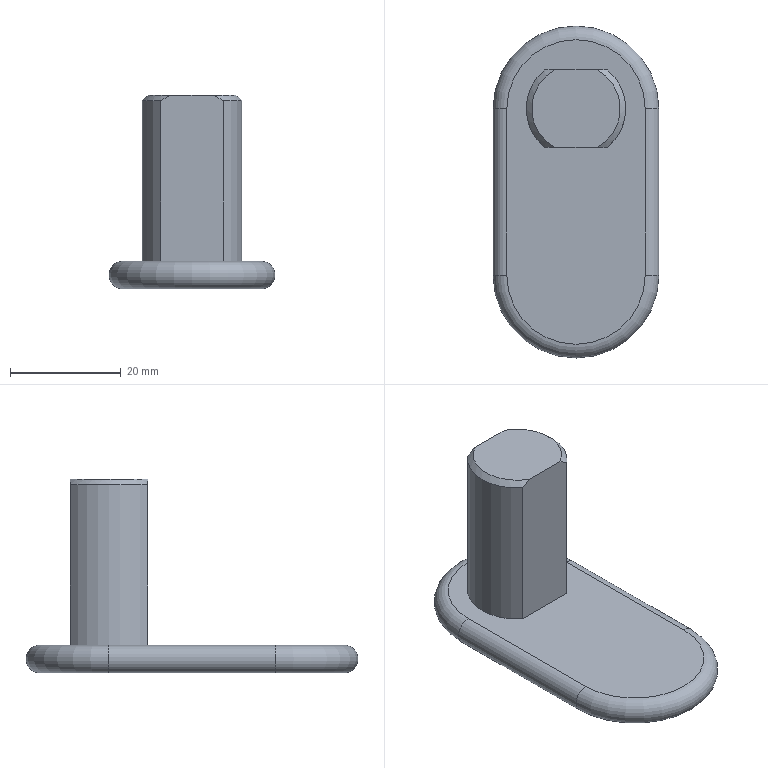Component | NX | LOWER_MOUNT | 1 solid | 13 faces | box 30 x 60 x 35 mm | volume 14320 mm3 | plane 5 | cylinder 4 | cone 2 | torus 2 | commonest cylinder face diameters 18 x2 5 x2
STEP:
#1=CARTESIAN_POINT('',(0.,0.,0.));
#2=DIRECTION('',(0.,0.,1.));
#3=DIRECTION('',(1.,0.,0.));
#4=AXIS2_PLACEMENT_3D('',#1,#2,#3);
#5=CARTESIAN_POINT('',(-12.5,94.875,-210.));
#6=VERTEX_POINT('',#5);
#7=CARTESIAN_POINT('',(12.5,94.875,-210.));
#8=VERTEX_POINT('',#7);
#9=CARTESIAN_POINT('',(0.,94.875,-210.));
#10=DIRECTION('',(0.,0.,1.));
#11=DIRECTION('',(0.,1.,0.));
#12=AXIS2_PLACEMENT_3D('',#9,#10,#11);
#13=CIRCLE('',#12,12.5);
#14=CARTESIAN_POINT('',(0.,94.875,-210.));
#15=DIRECTION('',(0.,0.,1.));
#16=DIRECTION('',(0.,1.,0.));
#17=AXIS2_PLACEMENT_3D('',#14,#15,#16);
#18=PLANE('',#17);
#19=CARTESIAN_POINT('',(0.,0.));
#20=DIRECTION('',(1.,0.));
#21=AXIS2_PLACEMENT_2D('',#19,#20);
#22=CIRCLE('',#21,12.5);
#23=(GEOMETRIC_REPRESENTATION_CONTEXT(2)PARAMETRIC_REPRESENTATION_CONTEXT()REPRESENTATION_CONTEXT('',''));
#24=DEFINITIONAL_REPRESENTATION('',(#22),#23);
#25=PCURVE('',#18,#24);
#26=CARTESIAN_POINT('',(0.,94.875,-212.5));
#27=DIRECTION('',(0.,0.,1.));
#28=DIRECTION('',(0.,1.,0.));
#29=AXIS2_PLACEMENT_3D('',#26,#27,#28);
#30=TOROIDAL_SURFACE('',#29,12.5,2.5);
#31=CARTESIAN_POINT('',(0.,7.854));
#32=DIRECTION('',(1.,0.));
#33=VECTOR('',#32,1.);
#34=LINE('',#31,#33);
#35=(GEOMETRIC_REPRESENTATION_CONTEXT(2)PARAMETRIC_REPRESENTATION_CONTEXT()REPRESENTATION_CONTEXT('',''));
#36=DEFINITIONAL_REPRESENTATION('',(#34),#35);
#37=PCURVE('',#30,#36);
#38=SURFACE_CURVE('',#13,(#25,#37),.PCURVE_S1.);
#39=EDGE_CURVE('',#6,#8,#38,.T.);
#40=ORIENTED_EDGE('',*,*,#39,.T.);
#41=CARTESIAN_POINT('',(12.5,124.875,-210.));
#42=VERTEX_POINT('',#41);
#43=CARTESIAN_POINT('',(12.5,94.875,-210.));
#44=DIRECTION('',(0.,1.,0.));
#45=VECTOR('',#44,1.);
#46=LINE('',#43,#45);
#47=CARTESIAN_POINT('',(0.,-12.5));
#48=DIRECTION('',(1.,0.));
#49=VECTOR('',#48,1.);
#50=LINE('',#47,#49);
#51=(GEOMETRIC_REPRESENTATION_CONTEXT(2)PARAMETRIC_REPRESENTATION_CONTEXT()REPRESENTATION_CONTEXT('',''));
#52=DEFINITIONAL_REPRESENTATION('',(#50),#51);
#53=PCURVE('',#18,#52);
#54=CARTESIAN_POINT('',(12.5,94.875,-212.5));
#55=DIRECTION('',(0.,-1.,0.));
#56=DIRECTION('',(0.,0.,1.));
#57=AXIS2_PLACEMENT_3D('',#54,#55,#56);
#58=CYLINDRICAL_SURFACE('',#57,2.5);
#59=CARTESIAN_POINT('',(6.283,0.));
#60=DIRECTION('',(0.,-1.));
#61=VECTOR('',#60,1.);
#62=LINE('',#59,#61);
#63=(GEOMETRIC_REPRESENTATION_CONTEXT(2)PARAMETRIC_REPRESENTATION_CONTEXT()REPRESENTATION_CONTEXT('',''));
#64=DEFINITIONAL_REPRESENTATION('',(#62),#63);
#65=PCURVE('',#58,#64);
#66=SURFACE_CURVE('',#46,(#53,#65),.PCURVE_S1.);
#67=EDGE_CURVE('',#8,#42,#66,.T.);
#68=ORIENTED_EDGE('',*,*,#67,.T.);
#69=CARTESIAN_POINT('',(-12.5,124.875,-210.));
#70=VERTEX_POINT('',#69);
#71=CARTESIAN_POINT('',(0.,124.875,-210.));
#72=DIRECTION('',(0.,0.,1.));
#73=DIRECTION('',(0.,1.,0.));
#74=AXIS2_PLACEMENT_3D('',#71,#72,#73);
#75=CIRCLE('',#74,12.5);
#76=CARTESIAN_POINT('',(30.,0.));
#77=DIRECTION('',(1.,0.));
#78=AXIS2_PLACEMENT_2D('',#76,#77);
#79=CIRCLE('',#78,12.5);
#80=(GEOMETRIC_REPRESENTATION_CONTEXT(2)PARAMETRIC_REPRESENTATION_CONTEXT()REPRESENTATION_CONTEXT('',''));
#81=DEFINITIONAL_REPRESENTATION('',(#79),#80);
#82=PCURVE('',#18,#81);
#83=CARTESIAN_POINT('',(0.,124.875,-212.5));
#84=DIRECTION('',(0.,0.,1.));
#85=DIRECTION('',(0.,1.,0.));
#86=AXIS2_PLACEMENT_3D('',#83,#84,#85);
#87=TOROIDAL_SURFACE('',#86,12.5,2.5);
#88=CARTESIAN_POINT('',(0.,7.854));
#89=DIRECTION('',(1.,0.));
#90=VECTOR('',#89,1.);
#91=LINE('',#88,#90);
#92=(GEOMETRIC_REPRESENTATION_CONTEXT(2)PARAMETRIC_REPRESENTATION_CONTEXT()REPRESENTATION_CONTEXT('',''));
#93=DEFINITIONAL_REPRESENTATION('',(#91),#92);
#94=PCURVE('',#87,#93);
#95=SURFACE_CURVE('',#75,(#82,#94),.PCURVE_S1.);
#96=EDGE_CURVE('',#42,#70,#95,.T.);
#97=ORIENTED_EDGE('',*,*,#96,.T.);
#98=CARTESIAN_POINT('',(-12.5,94.875,-210.));
#99=DIRECTION('',(0.,-1.,0.));
#100=VECTOR('',#99,1.);
#101=LINE('',#98,#100);
#102=CARTESIAN_POINT('',(0.,12.5));
#103=DIRECTION('',(-1.,0.));
#104=VECTOR('',#103,1.);
#105=LINE('',#102,#104);
#106=(GEOMETRIC_REPRESENTATION_CONTEXT(2)PARAMETRIC_REPRESENTATION_CONTEXT()REPRESENTATION_CONTEXT('',''));
#107=DEFINITIONAL_REPRESENTATION('',(#105),#106);
#108=PCURVE('',#18,#107);
#109=CARTESIAN_POINT('',(-12.5,124.875,-212.5));
#110=DIRECTION('',(0.,1.,0.));
#111=DIRECTION('',(0.,0.,-1.));
#112=AXIS2_PLACEMENT_3D('',#109,#110,#111);
#113=CYLINDRICAL_SURFACE('',#112,2.5);
#114=CARTESIAN_POINT('',(3.142,-30.));
#115=DIRECTION('',(0.,-1.));
#116=VECTOR('',#115,1.);
#117=LINE('',#114,#116);
#118=(GEOMETRIC_REPRESENTATION_CONTEXT(2)PARAMETRIC_REPRESENTATION_CONTEXT()REPRESENTATION_CONTEXT('',''));
#119=DEFINITIONAL_REPRESENTATION('',(#117),#118);
#120=PCURVE('',#113,#119);
#121=SURFACE_CURVE('',#101,(#108,#120),.PCURVE_S1.);
#122=EDGE_CURVE('',#70,#6,#121,.T.);
#123=ORIENTED_EDGE('',*,*,#122,.T.);
#124=EDGE_LOOP('',(#40,#68,#97,#123));
#125=FACE_BOUND('',#124,.T.);
#126=CARTESIAN_POINT('',(-5.657,117.875,-210.));
#127=VERTEX_POINT('',#126);
#128=CARTESIAN_POINT('',(5.657,117.875,-210.));
#129=VERTEX_POINT('',#128);
#130=CARTESIAN_POINT('',(0.,117.875,-210.));
#131=DIRECTION('',(1.,0.,0.));
#132=VECTOR('',#131,1.);
#133=LINE('',#130,#132);
#134=CARTESIAN_POINT('',(23.,0.));
#135=DIRECTION('',(0.,-1.));
#136=VECTOR('',#135,1.);
#137=LINE('',#134,#136);
#138=(GEOMETRIC_REPRESENTATION_CONTEXT(2)PARAMETRIC_REPRESENTATION_CONTEXT()REPRESENTATION_CONTEXT('',''));
#139=DEFINITIONAL_REPRESENTATION('',(#137),#138);
#140=PCURVE('',#18,#139);
#141=CARTESIAN_POINT('',(0.,117.875,-180.));
#142=DIRECTION('',(0.,-1.,0.));
#143=DIRECTION('',(0.,0.,1.));
#144=AXIS2_PLACEMENT_3D('',#141,#142,#143);
#145=PLANE('',#144);
#146=CARTESIAN_POINT('',(-30.,0.));
#147=DIRECTION('',(0.,-1.));
#148=VECTOR('',#147,1.);
#149=LINE('',#146,#148);
#150=(GEOMETRIC_REPRESENTATION_CONTEXT(2)PARAMETRIC_REPRESENTATION_CONTEXT()REPRESENTATION_CONTEXT('',''));
#151=DEFINITIONAL_REPRESENTATION('',(#149),#150);
#152=PCURVE('',#145,#151);
#153=SURFACE_CURVE('',#133,(#140,#152),.PCURVE_S1.);
#154=EDGE_CURVE('',#127,#129,#153,.T.);
#155=ORIENTED_EDGE('',*,*,#154,.F.);
#156=CARTESIAN_POINT('',(-5.657,131.875,-210.));
#157=VERTEX_POINT('',#156);
#158=CARTESIAN_POINT('',(0.,124.875,-210.));
#159=DIRECTION('',(0.,0.,1.));
#160=DIRECTION('',(0.,1.,0.));
#161=AXIS2_PLACEMENT_3D('',#158,#159,#160);
#162=CIRCLE('',#161,9.);
#163=CARTESIAN_POINT('',(30.,0.));
#164=DIRECTION('',(1.,0.));
#165=AXIS2_PLACEMENT_2D('',#163,#164);
#166=CIRCLE('',#165,9.);
#167=(GEOMETRIC_REPRESENTATION_CONTEXT(2)PARAMETRIC_REPRESENTATION_CONTEXT()REPRESENTATION_CONTEXT('',''));
#168=DEFINITIONAL_REPRESENTATION('',(#166),#167);
#169=PCURVE('',#18,#168);
#170=CARTESIAN_POINT('',(0.,124.875,-180.));
#171=DIRECTION('',(0.,0.,-1.));
#172=DIRECTION('',(0.,-1.,0.));
#173=AXIS2_PLACEMENT_3D('',#170,#171,#172);
#174=CYLINDRICAL_SURFACE('',#173,9.);
#175=CARTESIAN_POINT('',(3.142,30.));
#176=DIRECTION('',(-1.,0.));
#177=VECTOR('',#176,1.);
#178=LINE('',#175,#177);
#179=(GEOMETRIC_REPRESENTATION_CONTEXT(2)PARAMETRIC_REPRESENTATION_CONTEXT()REPRESENTATION_CONTEXT('',''));
#180=DEFINITIONAL_REPRESENTATION('',(#178),#179);
#181=PCURVE('',#174,#180);
#182=SURFACE_CURVE('',#162,(#169,#181),.PCURVE_S1.);
#183=EDGE_CURVE('',#157,#127,#182,.T.);
#184=ORIENTED_EDGE('',*,*,#183,.F.);
#185=CARTESIAN_POINT('',(5.657,131.875,-210.));
#186=VERTEX_POINT('',#185);
#187=CARTESIAN_POINT('',(0.,131.875,-210.));
#188=DIRECTION('',(-1.,0.,0.));
#189=VECTOR('',#188,1.);
#190=LINE('',#187,#189);
#191=CARTESIAN_POINT('',(37.,0.));
#192=DIRECTION('',(0.,1.));
#193=VECTOR('',#192,1.);
#194=LINE('',#191,#193);
#195=(GEOMETRIC_REPRESENTATION_CONTEXT(2)PARAMETRIC_REPRESENTATION_CONTEXT()REPRESENTATION_CONTEXT('',''));
#196=DEFINITIONAL_REPRESENTATION('',(#194),#195);
#197=PCURVE('',#18,#196);
#198=CARTESIAN_POINT('',(0.,131.875,-180.));
#199=DIRECTION('',(0.,1.,0.));
#200=DIRECTION('',(0.,0.,-1.));
#201=AXIS2_PLACEMENT_3D('',#198,#199,#200);
#202=PLANE('',#201);
#203=CARTESIAN_POINT('',(30.,0.));
#204=DIRECTION('',(0.,1.));
#205=VECTOR('',#204,1.);
#206=LINE('',#203,#205);
#207=(GEOMETRIC_REPRESENTATION_CONTEXT(2)PARAMETRIC_REPRESENTATION_CONTEXT()REPRESENTATION_CONTEXT('',''));
#208=DEFINITIONAL_REPRESENTATION('',(#206),#207);
#209=PCURVE('',#202,#208);
#210=SURFACE_CURVE('',#190,(#197,#209),.PCURVE_S1.);
#211=EDGE_CURVE('',#186,#157,#210,.T.);
#212=ORIENTED_EDGE('',*,*,#211,.F.);
#213=CARTESIAN_POINT('',(0.,124.875,-210.));
#214=DIRECTION('',(0.,0.,1.));
#215=DIRECTION('',(0.,1.,0.));
#216=AXIS2_PLACEMENT_3D('',#213,#214,#215);
#217=CIRCLE('',#216,9.);
#218=CARTESIAN_POINT('',(30.,0.));
#219=DIRECTION('',(1.,0.));
#220=AXIS2_PLACEMENT_2D('',#218,#219);
#221=CIRCLE('',#220,9.);
#222=(GEOMETRIC_REPRESENTATION_CONTEXT(2)PARAMETRIC_REPRESENTATION_CONTEXT()REPRESENTATION_CONTEXT('',''));
#223=DEFINITIONAL_REPRESENTATION('',(#221),#222);
#224=PCURVE('',#18,#223);
#225=CARTESIAN_POINT('',(0.,124.875,-180.));
#226=DIRECTION('',(0.,0.,-1.));
#227=DIRECTION('',(0.,-1.,0.));
#228=AXIS2_PLACEMENT_3D('',#225,#226,#227);
#229=CYLINDRICAL_SURFACE('',#228,9.);
#230=CARTESIAN_POINT('',(9.425,30.));
#231=DIRECTION('',(-1.,0.));
#232=VECTOR('',#231,1.);
#233=LINE('',#230,#232);
#234=(GEOMETRIC_REPRESENTATION_CONTEXT(2)PARAMETRIC_REPRESENTATION_CONTEXT()REPRESENTATION_CONTEXT('',''));
#235=DEFINITIONAL_REPRESENTATION('',(#233),#234);
#236=PCURVE('',#229,#235);
#237=SURFACE_CURVE('',#217,(#224,#236),.PCURVE_S1.);
#238=EDGE_CURVE('',#129,#186,#237,.T.);
#239=ORIENTED_EDGE('',*,*,#238,.F.);
#240=EDGE_LOOP('',(#155,#184,#212,#239));
#241=FACE_BOUND('',#240,.T.);
#242=ADVANCED_FACE('',(#125,#241),#18,.T.);
#243=CARTESIAN_POINT('',(-12.5,94.875,-215.));
#244=VERTEX_POINT('',#243);
#245=CARTESIAN_POINT('',(-12.5,124.875,-215.));
#246=VERTEX_POINT('',#245);
#247=CARTESIAN_POINT('',(-12.5,124.875,-215.));
#248=DIRECTION('',(0.,1.,0.));
#249=VECTOR('',#248,1.);
#250=LINE('',#247,#249);
#251=CARTESIAN_POINT('',(0.,94.875,-215.));
#252=DIRECTION('',(0.,0.,1.));
#253=DIRECTION('',(0.,1.,0.));
#254=AXIS2_PLACEMENT_3D('',#251,#252,#253);
#255=PLANE('',#254);
#256=CARTESIAN_POINT('',(30.,12.5));
#257=DIRECTION('',(1.,0.));
#258=VECTOR('',#257,1.);
#259=LINE('',#256,#258);
#260=(GEOMETRIC_REPRESENTATION_CONTEXT(2)PARAMETRIC_REPRESENTATION_CONTEXT()REPRESENTATION_CONTEXT('',''));
#261=DEFINITIONAL_REPRESENTATION('',(#259),#260);
#262=PCURVE('',#255,#261);
#263=CARTESIAN_POINT('',(0.,0.));
#264=DIRECTION('',(0.,1.));
#265=VECTOR('',#264,1.);
#266=LINE('',#263,#265);
#267=(GEOMETRIC_REPRESENTATION_CONTEXT(2)PARAMETRIC_REPRESENTATION_CONTEXT()REPRESENTATION_CONTEXT('',''));
#268=DEFINITIONAL_REPRESENTATION('',(#266),#267);
#269=PCURVE('',#113,#268);
#270=SURFACE_CURVE('',#250,(#262,#269),.PCURVE_S1.);
#271=EDGE_CURVE('',#244,#246,#270,.T.);
#272=ORIENTED_EDGE('',*,*,#271,.T.);
#273=CARTESIAN_POINT('',(12.5,124.875,-215.));
#274=VERTEX_POINT('',#273);
#275=CARTESIAN_POINT('',(0.,124.875,-215.));
#276=DIRECTION('',(0.,0.,-1.));
#277=DIRECTION('',(0.,1.,0.));
#278=AXIS2_PLACEMENT_3D('',#275,#276,#277);
#279=CIRCLE('',#278,12.5);
#280=CARTESIAN_POINT('',(42.5,0.));
#281=CARTESIAN_POINT('',(42.5,-21.651));
#282=CARTESIAN_POINT('',(23.75,-10.825));
#283=CARTESIAN_POINT('',(5.,-0.));
#284=CARTESIAN_POINT('',(23.75,10.825));
#285=CARTESIAN_POINT('',(42.5,21.651));
#286=CARTESIAN_POINT('',(42.5,0.));
#287=(BOUNDED_CURVE()B_SPLINE_CURVE(2,(#280,#281,#282,#283,#284,#285,#286),.UNSPECIFIED.,.T.,.F.)B_SPLINE_CURVE_WITH_KNOTS((1,2,2,2,2,1),(-2.094,0.,2.094,4.189,6.283,8.378),.UNSPECIFIED.)CURVE()GEOMETRIC_REPRESENTATION_ITEM()RATIONAL_B_SPLINE_CURVE((1.,0.5,1.,0.5,1.,0.5,1.))REPRESENTATION_ITEM(''));
#288=(GEOMETRIC_REPRESENTATION_CONTEXT(2)PARAMETRIC_REPRESENTATION_CONTEXT()REPRESENTATION_CONTEXT('',''));
#289=DEFINITIONAL_REPRESENTATION('',(#287),#288);
#290=PCURVE('',#255,#289);
#291=CARTESIAN_POINT('',(12.566,4.712));
#292=DIRECTION('',(-1.,0.));
#293=VECTOR('',#292,1.);
#294=LINE('',#291,#293);
#295=(GEOMETRIC_REPRESENTATION_CONTEXT(2)PARAMETRIC_REPRESENTATION_CONTEXT()REPRESENTATION_CONTEXT('',''));
#296=DEFINITIONAL_REPRESENTATION('',(#294),#295);
#297=PCURVE('',#87,#296);
#298=SURFACE_CURVE('',#279,(#290,#297),.PCURVE_S1.);
#299=EDGE_CURVE('',#246,#274,#298,.T.);
#300=ORIENTED_EDGE('',*,*,#299,.T.);
#301=CARTESIAN_POINT('',(12.5,94.875,-215.));
#302=VERTEX_POINT('',#301);
#303=CARTESIAN_POINT('',(12.5,94.875,-215.));
#304=DIRECTION('',(0.,-1.,0.));
#305=VECTOR('',#304,1.);
#306=LINE('',#303,#305);
#307=CARTESIAN_POINT('',(0.,-12.5));
#308=DIRECTION('',(-1.,0.));
#309=VECTOR('',#308,1.);
#310=LINE('',#307,#309);
#311=(GEOMETRIC_REPRESENTATION_CONTEXT(2)PARAMETRIC_REPRESENTATION_CONTEXT()REPRESENTATION_CONTEXT('',''));
#312=DEFINITIONAL_REPRESENTATION('',(#310),#311);
#313=PCURVE('',#255,#312);
#314=CARTESIAN_POINT('',(3.142,0.));
#315=DIRECTION('',(0.,1.));
#316=VECTOR('',#315,1.);
#317=LINE('',#314,#316);
#318=(GEOMETRIC_REPRESENTATION_CONTEXT(2)PARAMETRIC_REPRESENTATION_CONTEXT()REPRESENTATION_CONTEXT('',''));
#319=DEFINITIONAL_REPRESENTATION('',(#317),#318);
#320=PCURVE('',#58,#319);
#321=SURFACE_CURVE('',#306,(#313,#320),.PCURVE_S1.);
#322=EDGE_CURVE('',#274,#302,#321,.T.);
#323=ORIENTED_EDGE('',*,*,#322,.T.);
#324=CARTESIAN_POINT('',(0.,94.875,-215.));
#325=DIRECTION('',(0.,0.,-1.));
#326=DIRECTION('',(0.,1.,0.));
#327=AXIS2_PLACEMENT_3D('',#324,#325,#326);
#328=CIRCLE('',#327,12.5);
#329=CARTESIAN_POINT('',(12.5,0.));
#330=CARTESIAN_POINT('',(12.5,-21.651));
#331=CARTESIAN_POINT('',(-6.25,-10.825));
#332=CARTESIAN_POINT('',(-25.,-0.));
#333=CARTESIAN_POINT('',(-6.25,10.825));
#334=CARTESIAN_POINT('',(12.5,21.651));
#335=CARTESIAN_POINT('',(12.5,0.));
#336=(BOUNDED_CURVE()B_SPLINE_CURVE(2,(#329,#330,#331,#332,#333,#334,#335),.UNSPECIFIED.,.T.,.F.)B_SPLINE_CURVE_WITH_KNOTS((1,2,2,2,2,1),(-2.094,0.,2.094,4.189,6.283,8.378),.UNSPECIFIED.)CURVE()GEOMETRIC_REPRESENTATION_ITEM()RATIONAL_B_SPLINE_CURVE((1.,0.5,1.,0.5,1.,0.5,1.))REPRESENTATION_ITEM(''));
#337=(GEOMETRIC_REPRESENTATION_CONTEXT(2)PARAMETRIC_REPRESENTATION_CONTEXT()REPRESENTATION_CONTEXT('',''));
#338=DEFINITIONAL_REPRESENTATION('',(#336),#337);
#339=PCURVE('',#255,#338);
#340=CARTESIAN_POINT('',(6.283,4.712));
#341=DIRECTION('',(-1.,0.));
#342=VECTOR('',#341,1.);
#343=LINE('',#340,#342);
#344=(GEOMETRIC_REPRESENTATION_CONTEXT(2)PARAMETRIC_REPRESENTATION_CONTEXT()REPRESENTATION_CONTEXT('',''));
#345=DEFINITIONAL_REPRESENTATION('',(#343),#344);
#346=PCURVE('',#30,#345);
#347=SURFACE_CURVE('',#328,(#339,#346),.PCURVE_S1.);
#348=EDGE_CURVE('',#302,#244,#347,.T.);
#349=ORIENTED_EDGE('',*,*,#348,.T.);
#350=EDGE_LOOP('',(#272,#300,#323,#349));
#351=FACE_BOUND('',#350,.T.);
#352=ADVANCED_FACE('',(#351),#255,.F.);
#353=CARTESIAN_POINT('',(-5.657,117.875,-181.));
#354=VERTEX_POINT('',#353);
#355=CARTESIAN_POINT('',(-5.657,117.875,-180.));
#356=DIRECTION('',(0.,0.,-1.));
#357=VECTOR('',#356,1.);
#358=LINE('',#355,#357);
#359=CARTESIAN_POINT('',(0.6797,0.));
#360=DIRECTION('',(0.,1.));
#361=VECTOR('',#360,1.);
#362=LINE('',#359,#361);
#363=(GEOMETRIC_REPRESENTATION_CONTEXT(2)PARAMETRIC_REPRESENTATION_CONTEXT()REPRESENTATION_CONTEXT('',''));
#364=DEFINITIONAL_REPRESENTATION('',(#362),#363);
#365=PCURVE('',#174,#364);
#366=CARTESIAN_POINT('',(0.,5.657));
#367=DIRECTION('',(-1.,0.));
#368=VECTOR('',#367,1.);
#369=LINE('',#366,#368);
#370=(GEOMETRIC_REPRESENTATION_CONTEXT(2)PARAMETRIC_REPRESENTATION_CONTEXT()REPRESENTATION_CONTEXT('',''));
#371=DEFINITIONAL_REPRESENTATION('',(#369),#370);
#372=PCURVE('',#145,#371);
#373=SURFACE_CURVE('',#358,(#365,#372),.PCURVE_S1.);
#374=EDGE_CURVE('',#354,#127,#373,.T.);
#375=ORIENTED_EDGE('',*,*,#374,.F.);
#376=CARTESIAN_POINT('',(-5.657,131.875,-181.));
#377=VERTEX_POINT('',#376);
#378=CARTESIAN_POINT('',(0.,124.875,-181.));
#379=DIRECTION('',(0.,0.,-1.));
#380=DIRECTION('',(0.,1.,0.));
#381=AXIS2_PLACEMENT_3D('',#378,#379,#380);
#382=CIRCLE('',#381,9.);
#383=CARTESIAN_POINT('',(-3.142,1.));
#384=DIRECTION('',(1.,0.));
#385=VECTOR('',#384,1.);
#386=LINE('',#383,#385);
#387=(GEOMETRIC_REPRESENTATION_CONTEXT(2)PARAMETRIC_REPRESENTATION_CONTEXT()REPRESENTATION_CONTEXT('',''));
#388=DEFINITIONAL_REPRESENTATION('',(#386),#387);
#389=PCURVE('',#174,#388);
#390=CARTESIAN_POINT('',(0.,124.875,-180.));
#391=DIRECTION('',(0.,0.,-1.));
#392=DIRECTION('',(0.,-1.,0.));
#393=AXIS2_PLACEMENT_3D('',#390,#391,#392);
#394=CONICAL_SURFACE('',#393,8.,0.7854);
#395=CARTESIAN_POINT('',(-3.142,1.));
#396=DIRECTION('',(1.,0.));
#397=VECTOR('',#396,1.);
#398=LINE('',#395,#397);
#399=(GEOMETRIC_REPRESENTATION_CONTEXT(2)PARAMETRIC_REPRESENTATION_CONTEXT()REPRESENTATION_CONTEXT('',''));
#400=DEFINITIONAL_REPRESENTATION('',(#398),#399);
#401=PCURVE('',#394,#400);
#402=SURFACE_CURVE('',#382,(#389,#401),.PCURVE_S1.);
#403=EDGE_CURVE('',#354,#377,#402,.T.);
#404=ORIENTED_EDGE('',*,*,#403,.T.);
#405=CARTESIAN_POINT('',(-5.657,131.875,-180.));
#406=DIRECTION('',(0.,0.,1.));
#407=VECTOR('',#406,1.);
#408=LINE('',#405,#407);
#409=CARTESIAN_POINT('',(2.462,0.));
#410=DIRECTION('',(0.,-1.));
#411=VECTOR('',#410,1.);
#412=LINE('',#409,#411);
#413=(GEOMETRIC_REPRESENTATION_CONTEXT(2)PARAMETRIC_REPRESENTATION_CONTEXT()REPRESENTATION_CONTEXT('',''));
#414=DEFINITIONAL_REPRESENTATION('',(#412),#413);
#415=PCURVE('',#174,#414);
#416=CARTESIAN_POINT('',(0.,5.657));
#417=DIRECTION('',(-1.,0.));
#418=VECTOR('',#417,1.);
#419=LINE('',#416,#418);
#420=(GEOMETRIC_REPRESENTATION_CONTEXT(2)PARAMETRIC_REPRESENTATION_CONTEXT()REPRESENTATION_CONTEXT('',''));
#421=DEFINITIONAL_REPRESENTATION('',(#419),#420);
#422=PCURVE('',#202,#421);
#423=SURFACE_CURVE('',#408,(#415,#422),.PCURVE_S1.);
#424=EDGE_CURVE('',#157,#377,#423,.T.);
#425=ORIENTED_EDGE('',*,*,#424,.F.);
#426=ORIENTED_EDGE('',*,*,#183,.T.);
#427=EDGE_LOOP('',(#375,#404,#425,#426));
#428=FACE_BOUND('',#427,.T.);
#429=ADVANCED_FACE('',(#428),#174,.T.);
#430=CARTESIAN_POINT('',(5.657,117.875,-181.));
#431=VERTEX_POINT('',#430);
#432=CARTESIAN_POINT('',(5.657,117.875,-180.));
#433=DIRECTION('',(0.,0.,1.));
#434=VECTOR('',#433,1.);
#435=LINE('',#432,#434);
#436=CARTESIAN_POINT('',(5.604,0.));
#437=DIRECTION('',(0.,-1.));
#438=VECTOR('',#437,1.);
#439=LINE('',#436,#438);
#440=(GEOMETRIC_REPRESENTATION_CONTEXT(2)PARAMETRIC_REPRESENTATION_CONTEXT()REPRESENTATION_CONTEXT('',''));
#441=DEFINITIONAL_REPRESENTATION('',(#439),#440);
#442=PCURVE('',#229,#441);
#443=CARTESIAN_POINT('',(0.,-5.657));
#444=DIRECTION('',(1.,0.));
#445=VECTOR('',#444,1.);
#446=LINE('',#443,#445);
#447=(GEOMETRIC_REPRESENTATION_CONTEXT(2)PARAMETRIC_REPRESENTATION_CONTEXT()REPRESENTATION_CONTEXT('',''));
#448=DEFINITIONAL_REPRESENTATION('',(#446),#447);
#449=PCURVE('',#145,#448);
#450=SURFACE_CURVE('',#435,(#442,#449),.PCURVE_S1.);
#451=EDGE_CURVE('',#129,#431,#450,.T.);
#452=ORIENTED_EDGE('',*,*,#451,.F.);
#453=ORIENTED_EDGE('',*,*,#238,.T.);
#454=CARTESIAN_POINT('',(5.657,131.875,-181.));
#455=VERTEX_POINT('',#454);
#456=CARTESIAN_POINT('',(5.657,131.875,-180.));
#457=DIRECTION('',(0.,0.,-1.));
#458=VECTOR('',#457,1.);
#459=LINE('',#456,#458);
#460=CARTESIAN_POINT('',(3.821,0.));
#461=DIRECTION('',(0.,1.));
#462=VECTOR('',#461,1.);
#463=LINE('',#460,#462);
#464=(GEOMETRIC_REPRESENTATION_CONTEXT(2)PARAMETRIC_REPRESENTATION_CONTEXT()REPRESENTATION_CONTEXT('',''));
#465=DEFINITIONAL_REPRESENTATION('',(#463),#464);
#466=PCURVE('',#229,#465);
#467=CARTESIAN_POINT('',(0.,-5.657));
#468=DIRECTION('',(1.,0.));
#469=VECTOR('',#468,1.);
#470=LINE('',#467,#469);
#471=(GEOMETRIC_REPRESENTATION_CONTEXT(2)PARAMETRIC_REPRESENTATION_CONTEXT()REPRESENTATION_CONTEXT('',''));
#472=DEFINITIONAL_REPRESENTATION('',(#470),#471);
#473=PCURVE('',#202,#472);
#474=SURFACE_CURVE('',#459,(#466,#473),.PCURVE_S1.);
#475=EDGE_CURVE('',#455,#186,#474,.T.);
#476=ORIENTED_EDGE('',*,*,#475,.F.);
#477=CARTESIAN_POINT('',(0.,124.875,-181.));
#478=DIRECTION('',(0.,0.,-1.));
#479=DIRECTION('',(0.,1.,0.));
#480=AXIS2_PLACEMENT_3D('',#477,#478,#479);
#481=CIRCLE('',#480,9.);
#482=CARTESIAN_POINT('',(3.142,1.));
#483=DIRECTION('',(1.,0.));
#484=VECTOR('',#483,1.);
#485=LINE('',#482,#484);
#486=(GEOMETRIC_REPRESENTATION_CONTEXT(2)PARAMETRIC_REPRESENTATION_CONTEXT()REPRESENTATION_CONTEXT('',''));
#487=DEFINITIONAL_REPRESENTATION('',(#485),#486);
#488=PCURVE('',#229,#487);
#489=CARTESIAN_POINT('',(0.,124.875,-180.));
#490=DIRECTION('',(0.,0.,-1.));
#491=DIRECTION('',(0.,-1.,0.));
#492=AXIS2_PLACEMENT_3D('',#489,#490,#491);
#493=CONICAL_SURFACE('',#492,8.,0.7854);
#494=CARTESIAN_POINT('',(3.142,1.));
#495=DIRECTION('',(1.,0.));
#496=VECTOR('',#495,1.);
#497=LINE('',#494,#496);
#498=(GEOMETRIC_REPRESENTATION_CONTEXT(2)PARAMETRIC_REPRESENTATION_CONTEXT()REPRESENTATION_CONTEXT('',''));
#499=DEFINITIONAL_REPRESENTATION('',(#497),#498);
#500=PCURVE('',#493,#499);
#501=SURFACE_CURVE('',#481,(#488,#500),.PCURVE_S1.);
#502=EDGE_CURVE('',#455,#431,#501,.T.);
#503=ORIENTED_EDGE('',*,*,#502,.T.);
#504=EDGE_LOOP('',(#452,#453,#476,#503));
#505=FACE_BOUND('',#504,.T.);
#506=ADVANCED_FACE('',(#505),#229,.T.);
#507=CARTESIAN_POINT('',(-3.873,131.875,-180.));
#508=VERTEX_POINT('',#507);
#509=CARTESIAN_POINT('',(-3.873,117.875,-180.));
#510=VERTEX_POINT('',#509);
#511=CARTESIAN_POINT('',(0.,124.875,-180.));
#512=DIRECTION('',(0.,0.,1.));
#513=DIRECTION('',(0.,1.,0.));
#514=AXIS2_PLACEMENT_3D('',#511,#512,#513);
#515=CIRCLE('',#514,8.);
#516=CARTESIAN_POINT('',(0.,124.875,-180.));
#517=DIRECTION('',(0.,0.,1.));
#518=DIRECTION('',(0.,1.,0.));
#519=AXIS2_PLACEMENT_3D('',#516,#517,#518);
#520=PLANE('',#519);
#521=CARTESIAN_POINT('',(0.,0.));
#522=DIRECTION('',(1.,0.));
#523=AXIS2_PLACEMENT_2D('',#521,#522);
#524=CIRCLE('',#523,8.);
#525=(GEOMETRIC_REPRESENTATION_CONTEXT(2)PARAMETRIC_REPRESENTATION_CONTEXT()REPRESENTATION_CONTEXT('',''));
#526=DEFINITIONAL_REPRESENTATION('',(#524),#525);
#527=PCURVE('',#520,#526);
#528=CARTESIAN_POINT('',(3.142,0.));
#529=DIRECTION('',(-1.,-0.));
#530=VECTOR('',#529,1.);
#531=LINE('',#528,#530);
#532=(GEOMETRIC_REPRESENTATION_CONTEXT(2)PARAMETRIC_REPRESENTATION_CONTEXT()REPRESENTATION_CONTEXT('',''));
#533=DEFINITIONAL_REPRESENTATION('',(#531),#532);
#534=PCURVE('',#394,#533);
#535=SURFACE_CURVE('',#515,(#527,#534),.PCURVE_S1.);
#536=EDGE_CURVE('',#508,#510,#535,.T.);
#537=ORIENTED_EDGE('',*,*,#536,.T.);
#538=CARTESIAN_POINT('',(3.873,117.875,-180.));
#539=VERTEX_POINT('',#538);
#540=CARTESIAN_POINT('',(0.,117.875,-180.));
#541=DIRECTION('',(1.,0.,0.));
#542=VECTOR('',#541,1.);
#543=LINE('',#540,#542);
#544=CARTESIAN_POINT('',(-7.,0.));
#545=DIRECTION('',(0.,-1.));
#546=VECTOR('',#545,1.);
#547=LINE('',#544,#546);
#548=(GEOMETRIC_REPRESENTATION_CONTEXT(2)PARAMETRIC_REPRESENTATION_CONTEXT()REPRESENTATION_CONTEXT('',''));
#549=DEFINITIONAL_REPRESENTATION('',(#547),#548);
#550=PCURVE('',#520,#549);
#551=CARTESIAN_POINT('',(0.,0.));
#552=DIRECTION('',(0.,-1.));
#553=VECTOR('',#552,1.);
#554=LINE('',#551,#553);
#555=(GEOMETRIC_REPRESENTATION_CONTEXT(2)PARAMETRIC_REPRESENTATION_CONTEXT()REPRESENTATION_CONTEXT('',''));
#556=DEFINITIONAL_REPRESENTATION('',(#554),#555);
#557=PCURVE('',#145,#556);
#558=SURFACE_CURVE('',#543,(#550,#557),.PCURVE_S1.);
#559=EDGE_CURVE('',#510,#539,#558,.T.);
#560=ORIENTED_EDGE('',*,*,#559,.T.);
#561=CARTESIAN_POINT('',(3.873,131.875,-180.));
#562=VERTEX_POINT('',#561);
#563=CARTESIAN_POINT('',(0.,124.875,-180.));
#564=DIRECTION('',(0.,0.,1.));
#565=DIRECTION('',(0.,1.,0.));
#566=AXIS2_PLACEMENT_3D('',#563,#564,#565);
#567=CIRCLE('',#566,8.);
#568=CARTESIAN_POINT('',(0.,0.));
#569=DIRECTION('',(1.,0.));
#570=AXIS2_PLACEMENT_2D('',#568,#569);
#571=CIRCLE('',#570,8.);
#572=(GEOMETRIC_REPRESENTATION_CONTEXT(2)PARAMETRIC_REPRESENTATION_CONTEXT()REPRESENTATION_CONTEXT('',''));
#573=DEFINITIONAL_REPRESENTATION('',(#571),#572);
#574=PCURVE('',#520,#573);
#575=CARTESIAN_POINT('',(9.425,0.));
#576=DIRECTION('',(-1.,-0.));
#577=VECTOR('',#576,1.);
#578=LINE('',#575,#577);
#579=(GEOMETRIC_REPRESENTATION_CONTEXT(2)PARAMETRIC_REPRESENTATION_CONTEXT()REPRESENTATION_CONTEXT('',''));
#580=DEFINITIONAL_REPRESENTATION('',(#578),#579);
#581=PCURVE('',#493,#580);
#582=SURFACE_CURVE('',#567,(#574,#581),.PCURVE_S1.);
#583=EDGE_CURVE('',#539,#562,#582,.T.);
#584=ORIENTED_EDGE('',*,*,#583,.T.);
#585=CARTESIAN_POINT('',(0.,131.875,-180.));
#586=DIRECTION('',(-1.,0.,0.));
#587=VECTOR('',#586,1.);
#588=LINE('',#585,#587);
#589=CARTESIAN_POINT('',(7.,0.));
#590=DIRECTION('',(0.,1.));
#591=VECTOR('',#590,1.);
#592=LINE('',#589,#591);
#593=(GEOMETRIC_REPRESENTATION_CONTEXT(2)PARAMETRIC_REPRESENTATION_CONTEXT()REPRESENTATION_CONTEXT('',''));
#594=DEFINITIONAL_REPRESENTATION('',(#592),#593);
#595=PCURVE('',#520,#594);
#596=CARTESIAN_POINT('',(0.,0.));
#597=DIRECTION('',(0.,1.));
#598=VECTOR('',#597,1.);
#599=LINE('',#596,#598);
#600=(GEOMETRIC_REPRESENTATION_CONTEXT(2)PARAMETRIC_REPRESENTATION_CONTEXT()REPRESENTATION_CONTEXT('',''));
#601=DEFINITIONAL_REPRESENTATION('',(#599),#600);
#602=PCURVE('',#202,#601);
#603=SURFACE_CURVE('',#588,(#595,#602),.PCURVE_S1.);
#604=EDGE_CURVE('',#562,#508,#603,.T.);
#605=ORIENTED_EDGE('',*,*,#604,.T.);
#606=EDGE_LOOP('',(#537,#560,#584,#605));
#607=FACE_BOUND('',#606,.T.);
#608=ADVANCED_FACE('',(#607),#520,.T.);
#609=ORIENTED_EDGE('',*,*,#403,.F.);
#610=CARTESIAN_POINT('',(-5.657,117.875,-181.));
#611=CARTESIAN_POINT('',(-5.079,117.875,-180.637));
#612=CARTESIAN_POINT('',(-4.485,117.875,-180.296));
#613=CARTESIAN_POINT('',(-3.873,117.875,-180.));
#614=B_SPLINE_CURVE_WITH_KNOTS('',3,(#610,#611,#612,#613),.UNSPECIFIED.,.F.,.F.,(4,4),(0.,1.),.PIECEWISE_BEZIER_KNOTS.);
#615=CARTESIAN_POINT('',(0.6797,1.));
#616=CARTESIAN_POINT('',(0.6774,0.9835));
#617=CARTESIAN_POINT('',(0.6728,0.9506));
#618=CARTESIAN_POINT('',(0.6659,0.9015));
#619=CARTESIAN_POINT('',(0.6588,0.8527));
#620=CARTESIAN_POINT('',(0.6517,0.8042));
#621=CARTESIAN_POINT('',(0.6445,0.7561));
#622=CARTESIAN_POINT('',(0.6371,0.7083));
#623=CARTESIAN_POINT('',(0.6297,0.6609));
#624=CARTESIAN_POINT('',(0.6222,0.6139));
#625=CARTESIAN_POINT('',(0.6145,0.5672));
#626=CARTESIAN_POINT('',(0.6068,0.5209));
#627=CARTESIAN_POINT('',(0.5989,0.475));
#628=CARTESIAN_POINT('',(0.591,0.4295));
#629=CARTESIAN_POINT('',(0.5829,0.3844));
#630=CARTESIAN_POINT('',(0.5748,0.3398));
#631=CARTESIAN_POINT('',(0.5665,0.2956));
#632=CARTESIAN_POINT('',(0.5581,0.2519));
#633=CARTESIAN_POINT('',(0.5496,0.2087));
#634=CARTESIAN_POINT('',(0.541,0.1659));
#635=CARTESIAN_POINT('',(0.5323,0.1236));
#636=CARTESIAN_POINT('',(0.5234,0.08185));
#637=CARTESIAN_POINT('',(0.5145,0.04061));
#638=CARTESIAN_POINT('',(0.5084,0.01348));
#639=CARTESIAN_POINT('',(0.5054,0.));
#640=B_SPLINE_CURVE_WITH_KNOTS('',3,(#615,#616,#617,#618,#619,#620,#621,#622,#623,#624,#625,#626,#627,#628,#629,#630,#631,#632,#633,#634,#635,#636,#637,#638,#639),.UNSPECIFIED.,.F.,.F.,(4,1,1,1,1,1,1,1,1,1,1,1,1,1,1,1,1,1,1,1,1,1,4),(0.,0.04545,0.09091,0.1364,0.1818,0.2273,0.2727,0.3182,0.3636,0.4091,0.4545,0.5,0.5455,0.5909,0.6364,0.6818,0.7273,0.7727,0.8182,0.8636,0.9091,0.9545,1.),.QUASI_UNIFORM_KNOTS.);
#641=(GEOMETRIC_REPRESENTATION_CONTEXT(2)PARAMETRIC_REPRESENTATION_CONTEXT()REPRESENTATION_CONTEXT('',''));
#642=DEFINITIONAL_REPRESENTATION('',(#640),#641);
#643=PCURVE('',#394,#642);
#644=CARTESIAN_POINT('',(-1.,5.657));
#645=CARTESIAN_POINT('',(-0.6367,5.079));
#646=CARTESIAN_POINT('',(-0.2965,4.485));
#647=CARTESIAN_POINT('',(0.,3.873));
#648=B_SPLINE_CURVE_WITH_KNOTS('',3,(#644,#645,#646,#647),.UNSPECIFIED.,.F.,.F.,(4,4),(0.,1.),.PIECEWISE_BEZIER_KNOTS.);
#649=(GEOMETRIC_REPRESENTATION_CONTEXT(2)PARAMETRIC_REPRESENTATION_CONTEXT()REPRESENTATION_CONTEXT('',''));
#650=DEFINITIONAL_REPRESENTATION('',(#648),#649);
#651=PCURVE('',#145,#650);
#652=SURFACE_CURVE('',#614,(#643,#651),.PCURVE_S1.);
#653=EDGE_CURVE('',#354,#510,#652,.T.);
#654=ORIENTED_EDGE('',*,*,#653,.T.);
#655=ORIENTED_EDGE('',*,*,#536,.F.);
#656=CARTESIAN_POINT('',(-3.873,131.875,-180.));
#657=CARTESIAN_POINT('',(-4.488,131.875,-180.298));
#658=CARTESIAN_POINT('',(-5.079,131.875,-180.637));
#659=CARTESIAN_POINT('',(-5.657,131.875,-181.));
#660=B_SPLINE_CURVE_WITH_KNOTS('',3,(#656,#657,#658,#659),.UNSPECIFIED.,.F.,.F.,(4,4),(0.,1.),.PIECEWISE_BEZIER_KNOTS.);
#661=CARTESIAN_POINT('',(2.636,0.));
#662=CARTESIAN_POINT('',(2.633,0.01354));
#663=CARTESIAN_POINT('',(2.627,0.04079));
#664=CARTESIAN_POINT('',(2.618,0.08217));
#665=CARTESIAN_POINT('',(2.609,0.1241));
#666=CARTESIAN_POINT('',(2.6,0.1664));
#667=CARTESIAN_POINT('',(2.592,0.2093));
#668=CARTESIAN_POINT('',(2.583,0.2526));
#669=CARTESIAN_POINT('',(2.575,0.2963));
#670=CARTESIAN_POINT('',(2.567,0.3405));
#671=CARTESIAN_POINT('',(2.559,0.3851));
#672=CARTESIAN_POINT('',(2.55,0.4302));
#673=CARTESIAN_POINT('',(2.543,0.4756));
#674=CARTESIAN_POINT('',(2.535,0.5215));
#675=CARTESIAN_POINT('',(2.527,0.5677));
#676=CARTESIAN_POINT('',(2.519,0.6144));
#677=CARTESIAN_POINT('',(2.512,0.6614));
#678=CARTESIAN_POINT('',(2.504,0.7087));
#679=CARTESIAN_POINT('',(2.497,0.7564));
#680=CARTESIAN_POINT('',(2.49,0.8045));
#681=CARTESIAN_POINT('',(2.483,0.8529));
#682=CARTESIAN_POINT('',(2.476,0.9016));
#683=CARTESIAN_POINT('',(2.469,0.9506));
#684=CARTESIAN_POINT('',(2.464,0.9835));
#685=CARTESIAN_POINT('',(2.462,1.));
#686=B_SPLINE_CURVE_WITH_KNOTS('',3,(#661,#662,#663,#664,#665,#666,#667,#668,#669,#670,#671,#672,#673,#674,#675,#676,#677,#678,#679,#680,#681,#682,#683,#684,#685),.UNSPECIFIED.,.F.,.F.,(4,1,1,1,1,1,1,1,1,1,1,1,1,1,1,1,1,1,1,1,1,1,4),(0.,0.04545,0.09091,0.1364,0.1818,0.2273,0.2727,0.3182,0.3636,0.4091,0.4545,0.5,0.5455,0.5909,0.6364,0.6818,0.7273,0.7727,0.8182,0.8636,0.9091,0.9545,1.),.QUASI_UNIFORM_KNOTS.);
#687=(GEOMETRIC_REPRESENTATION_CONTEXT(2)PARAMETRIC_REPRESENTATION_CONTEXT()REPRESENTATION_CONTEXT('',''));
#688=DEFINITIONAL_REPRESENTATION('',(#686),#687);
#689=PCURVE('',#394,#688);
#690=CARTESIAN_POINT('',(0.,3.873));
#691=CARTESIAN_POINT('',(0.2978,4.488));
#692=CARTESIAN_POINT('',(0.637,5.079));
#693=CARTESIAN_POINT('',(1.,5.657));
#694=B_SPLINE_CURVE_WITH_KNOTS('',3,(#690,#691,#692,#693),.UNSPECIFIED.,.F.,.F.,(4,4),(0.,1.),.PIECEWISE_BEZIER_KNOTS.);
#695=(GEOMETRIC_REPRESENTATION_CONTEXT(2)PARAMETRIC_REPRESENTATION_CONTEXT()REPRESENTATION_CONTEXT('',''));
#696=DEFINITIONAL_REPRESENTATION('',(#694),#695);
#697=PCURVE('',#202,#696);
#698=SURFACE_CURVE('',#660,(#689,#697),.PCURVE_S1.);
#699=EDGE_CURVE('',#508,#377,#698,.T.);
#700=ORIENTED_EDGE('',*,*,#699,.T.);
#701=EDGE_LOOP('',(#609,#654,#655,#700));
#702=FACE_BOUND('',#701,.T.);
#703=ADVANCED_FACE('',(#702),#394,.T.);
#704=ORIENTED_EDGE('',*,*,#583,.F.);
#705=CARTESIAN_POINT('',(3.873,117.875,-180.));
#706=CARTESIAN_POINT('',(4.488,117.875,-180.298));
#707=CARTESIAN_POINT('',(5.079,117.875,-180.637));
#708=CARTESIAN_POINT('',(5.657,117.875,-181.));
#709=B_SPLINE_CURVE_WITH_KNOTS('',3,(#705,#706,#707,#708),.UNSPECIFIED.,.F.,.F.,(4,4),(0.,1.),.PIECEWISE_BEZIER_KNOTS.);
#710=CARTESIAN_POINT('',(5.778,0.));
#711=CARTESIAN_POINT('',(5.775,0.01354));
#712=CARTESIAN_POINT('',(5.769,0.04079));
#713=CARTESIAN_POINT('',(5.76,0.08217));
#714=CARTESIAN_POINT('',(5.751,0.1241));
#715=CARTESIAN_POINT('',(5.742,0.1664));
#716=CARTESIAN_POINT('',(5.733,0.2093));
#717=CARTESIAN_POINT('',(5.725,0.2526));
#718=CARTESIAN_POINT('',(5.717,0.2963));
#719=CARTESIAN_POINT('',(5.708,0.3405));
#720=CARTESIAN_POINT('',(5.7,0.3851));
#721=CARTESIAN_POINT('',(5.692,0.4302));
#722=CARTESIAN_POINT('',(5.684,0.4756));
#723=CARTESIAN_POINT('',(5.676,0.5215));
#724=CARTESIAN_POINT('',(5.669,0.5677));
#725=CARTESIAN_POINT('',(5.661,0.6144));
#726=CARTESIAN_POINT('',(5.653,0.6614));
#727=CARTESIAN_POINT('',(5.646,0.7087));
#728=CARTESIAN_POINT('',(5.639,0.7564));
#729=CARTESIAN_POINT('',(5.631,0.8045));
#730=CARTESIAN_POINT('',(5.624,0.8529));
#731=CARTESIAN_POINT('',(5.617,0.9016));
#732=CARTESIAN_POINT('',(5.61,0.9506));
#733=CARTESIAN_POINT('',(5.606,0.9835));
#734=CARTESIAN_POINT('',(5.604,1.));
#735=B_SPLINE_CURVE_WITH_KNOTS('',3,(#710,#711,#712,#713,#714,#715,#716,#717,#718,#719,#720,#721,#722,#723,#724,#725,#726,#727,#728,#729,#730,#731,#732,#733,#734),.UNSPECIFIED.,.F.,.F.,(4,1,1,1,1,1,1,1,1,1,1,1,1,1,1,1,1,1,1,1,1,1,4),(0.,0.04545,0.09091,0.1364,0.1818,0.2273,0.2727,0.3182,0.3636,0.4091,0.4545,0.5,0.5455,0.5909,0.6364,0.6818,0.7273,0.7727,0.8182,0.8636,0.9091,0.9545,1.),.QUASI_UNIFORM_KNOTS.);
#736=(GEOMETRIC_REPRESENTATION_CONTEXT(2)PARAMETRIC_REPRESENTATION_CONTEXT()REPRESENTATION_CONTEXT('',''));
#737=DEFINITIONAL_REPRESENTATION('',(#735),#736);
#738=PCURVE('',#493,#737);
#739=CARTESIAN_POINT('',(0.,-3.873));
#740=CARTESIAN_POINT('',(-0.2978,-4.488));
#741=CARTESIAN_POINT('',(-0.637,-5.079));
#742=CARTESIAN_POINT('',(-1.,-5.657));
#743=B_SPLINE_CURVE_WITH_KNOTS('',3,(#739,#740,#741,#742),.UNSPECIFIED.,.F.,.F.,(4,4),(0.,1.),.PIECEWISE_BEZIER_KNOTS.);
#744=(GEOMETRIC_REPRESENTATION_CONTEXT(2)PARAMETRIC_REPRESENTATION_CONTEXT()REPRESENTATION_CONTEXT('',''));
#745=DEFINITIONAL_REPRESENTATION('',(#743),#744);
#746=PCURVE('',#145,#745);
#747=SURFACE_CURVE('',#709,(#738,#746),.PCURVE_S1.);
#748=EDGE_CURVE('',#539,#431,#747,.T.);
#749=ORIENTED_EDGE('',*,*,#748,.T.);
#750=ORIENTED_EDGE('',*,*,#502,.F.);
#751=CARTESIAN_POINT('',(5.657,131.875,-181.));
#752=CARTESIAN_POINT('',(5.079,131.875,-180.637));
#753=CARTESIAN_POINT('',(4.485,131.875,-180.296));
#754=CARTESIAN_POINT('',(3.873,131.875,-180.));
#755=B_SPLINE_CURVE_WITH_KNOTS('',3,(#751,#752,#753,#754),.UNSPECIFIED.,.F.,.F.,(4,4),(0.,1.),.PIECEWISE_BEZIER_KNOTS.);
#756=CARTESIAN_POINT('',(3.821,1.));
#757=CARTESIAN_POINT('',(3.819,0.9835));
#758=CARTESIAN_POINT('',(3.814,0.9506));
#759=CARTESIAN_POINT('',(3.807,0.9015));
#760=CARTESIAN_POINT('',(3.8,0.8527));
#761=CARTESIAN_POINT('',(3.793,0.8042));
#762=CARTESIAN_POINT('',(3.786,0.7561));
#763=CARTESIAN_POINT('',(3.779,0.7083));
#764=CARTESIAN_POINT('',(3.771,0.6609));
#765=CARTESIAN_POINT('',(3.764,0.6139));
#766=CARTESIAN_POINT('',(3.756,0.5672));
#767=CARTESIAN_POINT('',(3.748,0.5209));
#768=CARTESIAN_POINT('',(3.741,0.475));
#769=CARTESIAN_POINT('',(3.733,0.4295));
#770=CARTESIAN_POINT('',(3.725,0.3844));
#771=CARTESIAN_POINT('',(3.716,0.3398));
#772=CARTESIAN_POINT('',(3.708,0.2956));
#773=CARTESIAN_POINT('',(3.7,0.2519));
#774=CARTESIAN_POINT('',(3.691,0.2087));
#775=CARTESIAN_POINT('',(3.683,0.1659));
#776=CARTESIAN_POINT('',(3.674,0.1236));
#777=CARTESIAN_POINT('',(3.665,0.08185));
#778=CARTESIAN_POINT('',(3.656,0.04061));
#779=CARTESIAN_POINT('',(3.65,0.01348));
#780=CARTESIAN_POINT('',(3.647,0.));
#781=B_SPLINE_CURVE_WITH_KNOTS('',3,(#756,#757,#758,#759,#760,#761,#762,#763,#764,#765,#766,#767,#768,#769,#770,#771,#772,#773,#774,#775,#776,#777,#778,#779,#780),.UNSPECIFIED.,.F.,.F.,(4,1,1,1,1,1,1,1,1,1,1,1,1,1,1,1,1,1,1,1,1,1,4),(0.,0.04545,0.09091,0.1364,0.1818,0.2273,0.2727,0.3182,0.3636,0.4091,0.4545,0.5,0.5455,0.5909,0.6364,0.6818,0.7273,0.7727,0.8182,0.8636,0.9091,0.9545,1.),.QUASI_UNIFORM_KNOTS.);
#782=(GEOMETRIC_REPRESENTATION_CONTEXT(2)PARAMETRIC_REPRESENTATION_CONTEXT()REPRESENTATION_CONTEXT('',''));
#783=DEFINITIONAL_REPRESENTATION('',(#781),#782);
#784=PCURVE('',#493,#783);
#785=CARTESIAN_POINT('',(1.,-5.657));
#786=CARTESIAN_POINT('',(0.6367,-5.079));
#787=CARTESIAN_POINT('',(0.2965,-4.485));
#788=CARTESIAN_POINT('',(0.,-3.873));
#789=B_SPLINE_CURVE_WITH_KNOTS('',3,(#785,#786,#787,#788),.UNSPECIFIED.,.F.,.F.,(4,4),(0.,1.),.PIECEWISE_BEZIER_KNOTS.);
#790=(GEOMETRIC_REPRESENTATION_CONTEXT(2)PARAMETRIC_REPRESENTATION_CONTEXT()REPRESENTATION_CONTEXT('',''));
#791=DEFINITIONAL_REPRESENTATION('',(#789),#790);
#792=PCURVE('',#202,#791);
#793=SURFACE_CURVE('',#755,(#784,#792),.PCURVE_S1.);
#794=EDGE_CURVE('',#455,#562,#793,.T.);
#795=ORIENTED_EDGE('',*,*,#794,.T.);
#796=EDGE_LOOP('',(#704,#749,#750,#795));
#797=FACE_BOUND('',#796,.T.);
#798=ADVANCED_FACE('',(#797),#493,.T.);
#799=ORIENTED_EDGE('',*,*,#794,.F.);
#800=ORIENTED_EDGE('',*,*,#475,.T.);
#801=ORIENTED_EDGE('',*,*,#211,.T.);
#802=ORIENTED_EDGE('',*,*,#424,.T.);
#803=ORIENTED_EDGE('',*,*,#699,.F.);
#804=ORIENTED_EDGE('',*,*,#604,.F.);
#805=EDGE_LOOP('',(#799,#800,#801,#802,#803,#804));
#806=FACE_BOUND('',#805,.T.);
#807=ADVANCED_FACE('',(#806),#202,.T.);
#808=ORIENTED_EDGE('',*,*,#653,.F.);
#809=ORIENTED_EDGE('',*,*,#374,.T.);
#810=ORIENTED_EDGE('',*,*,#154,.T.);
#811=ORIENTED_EDGE('',*,*,#451,.T.);
#812=ORIENTED_EDGE('',*,*,#748,.F.);
#813=ORIENTED_EDGE('',*,*,#559,.F.);
#814=EDGE_LOOP('',(#808,#809,#810,#811,#812,#813));
#815=FACE_BOUND('',#814,.T.);
#816=ADVANCED_FACE('',(#815),#145,.T.);
#817=CARTESIAN_POINT('',(12.5,94.875,-212.5));
#818=DIRECTION('',(0.,1.,0.));
#819=DIRECTION('',(0.,0.,-1.));
#820=AXIS2_PLACEMENT_3D('',#817,#818,#819);
#821=CIRCLE('',#820,2.5);
#822=CARTESIAN_POINT('',(4.712,10.996));
#823=DIRECTION('',(0.,-1.));
#824=VECTOR('',#823,1.);
#825=LINE('',#822,#824);
#826=(GEOMETRIC_REPRESENTATION_CONTEXT(2)PARAMETRIC_REPRESENTATION_CONTEXT()REPRESENTATION_CONTEXT('',''));
#827=DEFINITIONAL_REPRESENTATION('',(#825),#826);
#828=PCURVE('',#30,#827);
#829=CARTESIAN_POINT('',(9.425,0.));
#830=DIRECTION('',(-1.,0.));
#831=VECTOR('',#830,1.);
#832=LINE('',#829,#831);
#833=(GEOMETRIC_REPRESENTATION_CONTEXT(2)PARAMETRIC_REPRESENTATION_CONTEXT()REPRESENTATION_CONTEXT('',''));
#834=DEFINITIONAL_REPRESENTATION('',(#832),#833);
#835=PCURVE('',#58,#834);
#836=SURFACE_CURVE('',#821,(#828,#835),.PCURVE_S1.);
#837=EDGE_CURVE('',#8,#302,#836,.T.);
#838=ORIENTED_EDGE('',*,*,#837,.F.);
#839=ORIENTED_EDGE('',*,*,#39,.F.);
#840=CARTESIAN_POINT('',(-12.5,94.875,-212.5));
#841=DIRECTION('',(0.,1.,0.));
#842=DIRECTION('',(0.,0.,-1.));
#843=AXIS2_PLACEMENT_3D('',#840,#841,#842);
#844=CIRCLE('',#843,2.5);
#845=CARTESIAN_POINT('',(1.571,4.712));
#846=DIRECTION('',(0.,1.));
#847=VECTOR('',#846,1.);
#848=LINE('',#845,#847);
#849=(GEOMETRIC_REPRESENTATION_CONTEXT(2)PARAMETRIC_REPRESENTATION_CONTEXT()REPRESENTATION_CONTEXT('',''));
#850=DEFINITIONAL_REPRESENTATION('',(#848),#849);
#851=PCURVE('',#30,#850);
#852=CARTESIAN_POINT('',(0.,-30.));
#853=DIRECTION('',(1.,0.));
#854=VECTOR('',#853,1.);
#855=LINE('',#852,#854);
#856=(GEOMETRIC_REPRESENTATION_CONTEXT(2)PARAMETRIC_REPRESENTATION_CONTEXT()REPRESENTATION_CONTEXT('',''));
#857=DEFINITIONAL_REPRESENTATION('',(#855),#856);
#858=PCURVE('',#113,#857);
#859=SURFACE_CURVE('',#844,(#851,#858),.PCURVE_S1.);
#860=EDGE_CURVE('',#244,#6,#859,.T.);
#861=ORIENTED_EDGE('',*,*,#860,.F.);
#862=ORIENTED_EDGE('',*,*,#348,.F.);
#863=EDGE_LOOP('',(#838,#839,#861,#862));
#864=FACE_BOUND('',#863,.T.);
#865=ADVANCED_FACE('',(#864),#30,.T.);
#866=ORIENTED_EDGE('',*,*,#860,.T.);
#867=ORIENTED_EDGE('',*,*,#122,.F.);
#868=CARTESIAN_POINT('',(-12.5,124.875,-212.5));
#869=DIRECTION('',(0.,1.,0.));
#870=DIRECTION('',(0.,0.,-1.));
#871=AXIS2_PLACEMENT_3D('',#868,#869,#870);
#872=CIRCLE('',#871,2.5);
#873=CARTESIAN_POINT('',(0.,0.));
#874=DIRECTION('',(1.,0.));
#875=VECTOR('',#874,1.);
#876=LINE('',#873,#875);
#877=(GEOMETRIC_REPRESENTATION_CONTEXT(2)PARAMETRIC_REPRESENTATION_CONTEXT()REPRESENTATION_CONTEXT('',''));
#878=DEFINITIONAL_REPRESENTATION('',(#876),#877);
#879=PCURVE('',#113,#878);
#880=CARTESIAN_POINT('',(7.854,4.712));
#881=DIRECTION('',(0.,1.));
#882=VECTOR('',#881,1.);
#883=LINE('',#880,#882);
#884=(GEOMETRIC_REPRESENTATION_CONTEXT(2)PARAMETRIC_REPRESENTATION_CONTEXT()REPRESENTATION_CONTEXT('',''));
#885=DEFINITIONAL_REPRESENTATION('',(#883),#884);
#886=PCURVE('',#87,#885);
#887=SURFACE_CURVE('',#872,(#879,#886),.PCURVE_S1.);
#888=EDGE_CURVE('',#246,#70,#887,.T.);
#889=ORIENTED_EDGE('',*,*,#888,.F.);
#890=ORIENTED_EDGE('',*,*,#271,.F.);
#891=EDGE_LOOP('',(#866,#867,#889,#890));
#892=FACE_BOUND('',#891,.T.);
#893=ADVANCED_FACE('',(#892),#113,.T.);
#894=CARTESIAN_POINT('',(12.5,124.875,-212.5));
#895=DIRECTION('',(0.,1.,0.));
#896=DIRECTION('',(0.,0.,-1.));
#897=AXIS2_PLACEMENT_3D('',#894,#895,#896);
#898=CIRCLE('',#897,2.5);
#899=CARTESIAN_POINT('',(9.425,-30.));
#900=DIRECTION('',(-1.,0.));
#901=VECTOR('',#900,1.);
#902=LINE('',#899,#901);
#903=(GEOMETRIC_REPRESENTATION_CONTEXT(2)PARAMETRIC_REPRESENTATION_CONTEXT()REPRESENTATION_CONTEXT('',''));
#904=DEFINITIONAL_REPRESENTATION('',(#902),#903);
#905=PCURVE('',#58,#904);
#906=CARTESIAN_POINT('',(4.712,10.996));
#907=DIRECTION('',(0.,-1.));
#908=VECTOR('',#907,1.);
#909=LINE('',#906,#908);
#910=(GEOMETRIC_REPRESENTATION_CONTEXT(2)PARAMETRIC_REPRESENTATION_CONTEXT()REPRESENTATION_CONTEXT('',''));
#911=DEFINITIONAL_REPRESENTATION('',(#909),#910);
#912=PCURVE('',#87,#911);
#913=SURFACE_CURVE('',#898,(#905,#912),.PCURVE_S1.);
#914=EDGE_CURVE('',#42,#274,#913,.T.);
#915=ORIENTED_EDGE('',*,*,#914,.F.);
#916=ORIENTED_EDGE('',*,*,#67,.F.);
#917=ORIENTED_EDGE('',*,*,#837,.T.);
#918=ORIENTED_EDGE('',*,*,#322,.F.);
#919=EDGE_LOOP('',(#915,#916,#917,#918));
#920=FACE_BOUND('',#919,.T.);
#921=ADVANCED_FACE('',(#920),#58,.T.);
#922=ORIENTED_EDGE('',*,*,#96,.F.);
#923=ORIENTED_EDGE('',*,*,#914,.T.);
#924=ORIENTED_EDGE('',*,*,#299,.F.);
#925=ORIENTED_EDGE('',*,*,#888,.T.);
#926=EDGE_LOOP('',(#922,#923,#924,#925));
#927=FACE_BOUND('',#926,.T.);
#928=ADVANCED_FACE('',(#927),#87,.T.);
#929=CLOSED_SHELL('',(#242,#352,#429,#506,#608,#703,#798,#807,#816,#865,#893,#921,#928));
#930=MANIFOLD_SOLID_BREP('',#929);
#931=(LENGTH_UNIT()NAMED_UNIT(*)SI_UNIT(.MILLI.,.METRE.));
#932=UNCERTAINTY_MEASURE_WITH_UNIT(LENGTH_MEASURE(0.00005),#931,'','');
#933=(NAMED_UNIT(*)PLANE_ANGLE_UNIT()SI_UNIT($,.RADIAN.));
#934=(NAMED_UNIT(*)SI_UNIT($,.STERADIAN.)SOLID_ANGLE_UNIT());
#935=(GEOMETRIC_REPRESENTATION_CONTEXT(3)GLOBAL_UNCERTAINTY_ASSIGNED_CONTEXT((#932))GLOBAL_UNIT_ASSIGNED_CONTEXT((#931,#933,#934))REPRESENTATION_CONTEXT('',''));
#936=ADVANCED_BREP_SHAPE_REPRESENTATION('',(#4,#930),#935);